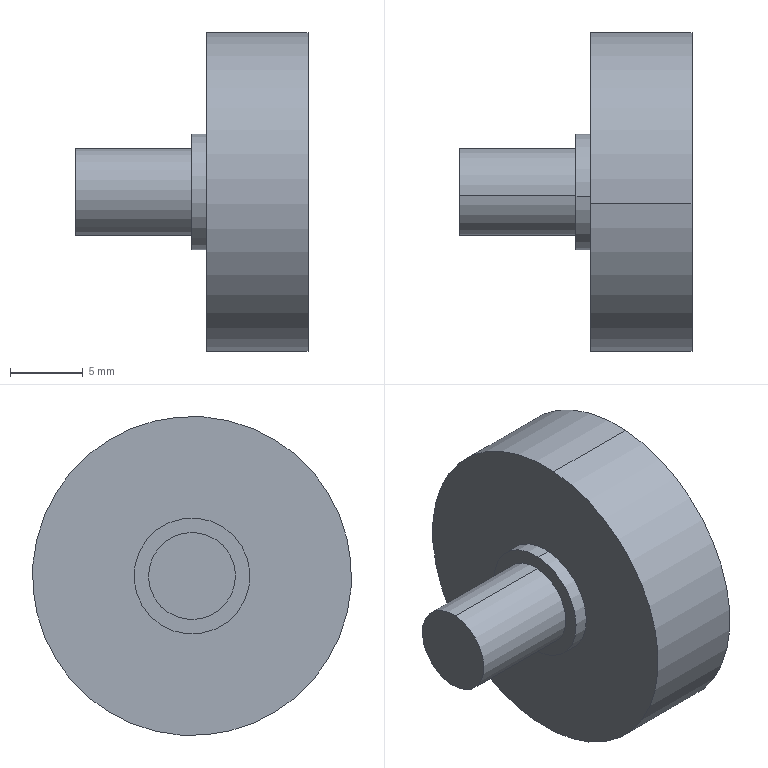Component | SolidWorks | JS60822-7C1L8M6ExternalThreadBearing-1 | 1 solid | 10 faces | box 16 x 22 x 22 mm | volume 2937 mm3 | cylinder 6 | plane 4 | commonest cylinder face diameters 6 x2 8 x2 22 x2
build123d program:
from build123d import *

# Parameters (mm, degrees)
SKETCH1_R           = 11
BOSS_EXTRUDE1_DEPTH = 7
SKETCH2_R           = 4
BOSS_EXTRUDE2_DEPTH = 1
SKETCH3_R           = 3
BOSS_EXTRUDE3_DEPTH = 8


with BuildPart() as part:
    # Sketch1 → Boss-Extrude1 (new body)
    with BuildSketch(Plane(origin=(0, 0, 0), x_dir=(0, 0, -1), z_dir=(1, 0, 0))):
        Circle(SKETCH1_R)
    extrude(amount=BOSS_EXTRUDE1_DEPTH)

    # Sketch2 → Boss-Extrude2 (add)
    with BuildSketch(Plane(origin=(7, 0, 0), x_dir=(0, 0, -1), z_dir=(1, 0, 0))):
        Circle(SKETCH2_R)
    extrude(amount=BOSS_EXTRUDE2_DEPTH)

    # Sketch3 → Boss-Extrude3 (add)
    with BuildSketch(Plane(origin=(8, 0, 0), x_dir=(0, 0, -1), z_dir=(1, 0, 0))):
        Circle(SKETCH3_R)
    extrude(amount=BOSS_EXTRUDE3_DEPTH)


solid = part.part

# Placed as in the assembly
solid = solid.moved(Location((234, 20, 79.212), (-180, 0, 180)))
STEP:
#1=COLOUR_RGB('',0.7922,0.8196,0.9333);
#2=FILL_AREA_STYLE_COLOUR('',#1);
#3=FILL_AREA_STYLE('',(#2));
#4=SURFACE_STYLE_FILL_AREA(#3);
#5=SURFACE_SIDE_STYLE('',(#4));
#6=SURFACE_STYLE_USAGE(.BOTH.,#5);
#7=PRESENTATION_STYLE_ASSIGNMENT((#6));
#8=CARTESIAN_POINT('',(8.583,0.7786,3.236));
#9=VERTEX_POINT('',#8);
#10=CARTESIAN_POINT('',(8.583,0.7962,3.001));
#11=VERTEX_POINT('',#10);
#12=CARTESIAN_POINT('',(8.583,0.7874,3.119));
#13=DIRECTION('',(-1.,-0.,0.));
#14=DIRECTION('',(0.,-0.07456,0.9972));
#15=AXIS2_PLACEMENT_3D('',#12,#13,#14);
#16=CIRCLE('',#15,0.1181);
#17=EDGE_CURVE('',#9,#11,#16,.T.);
#18=ORIENTED_EDGE('',*,*,#17,.F.);
#19=CARTESIAN_POINT('',(8.898,0.7786,3.236));
#20=VERTEX_POINT('',#19);
#21=CARTESIAN_POINT('',(8.583,0.7786,3.236));
#22=DIRECTION('',(1.,0.,0.));
#23=VECTOR('',#22,39.37);
#24=LINE('',#21,#23);
#25=EDGE_CURVE('',#9,#20,#24,.T.);
#26=ORIENTED_EDGE('',*,*,#25,.T.);
#27=CARTESIAN_POINT('',(8.898,0.7962,3.001));
#28=VERTEX_POINT('',#27);
#29=CARTESIAN_POINT('',(8.898,0.7874,3.119));
#30=DIRECTION('',(-1.,-0.,0.));
#31=DIRECTION('',(0.,-0.07456,0.9972));
#32=AXIS2_PLACEMENT_3D('',#29,#30,#31);
#33=CIRCLE('',#32,0.1181);
#34=EDGE_CURVE('',#20,#28,#33,.T.);
#35=ORIENTED_EDGE('',*,*,#34,.T.);
#36=CARTESIAN_POINT('',(8.583,0.7962,3.001));
#37=DIRECTION('',(1.,0.,0.));
#38=VECTOR('',#37,39.37);
#39=LINE('',#36,#38);
#40=EDGE_CURVE('',#11,#28,#39,.T.);
#41=ORIENTED_EDGE('',*,*,#40,.F.);
#42=EDGE_LOOP('',(#18,#26,#35,#41));
#43=FACE_OUTER_BOUND('',#42,.T.);
#44=CARTESIAN_POINT('',(8.583,0.7874,3.119));
#45=DIRECTION('',(1.,0.,0.));
#46=DIRECTION('',(0.,0.07456,-0.9972));
#47=AXIS2_PLACEMENT_3D('',#44,#45,#46);
#48=CYLINDRICAL_SURFACE('',#47,0.1181);
#49=ADVANCED_FACE('',(#43),#48,.T.);
#50=CARTESIAN_POINT('',(8.898,0.7757,3.276));
#51=VERTEX_POINT('',#50);
#52=CARTESIAN_POINT('',(8.898,0.7991,2.962));
#53=VERTEX_POINT('',#52);
#54=CARTESIAN_POINT('',(8.898,0.7874,3.119));
#55=DIRECTION('',(-1.,-0.,0.));
#56=DIRECTION('',(0.,-0.07456,0.9972));
#57=AXIS2_PLACEMENT_3D('',#54,#55,#56);
#58=CIRCLE('',#57,0.1575);
#59=EDGE_CURVE('',#51,#53,#58,.T.);
#60=ORIENTED_EDGE('',*,*,#59,.F.);
#61=CARTESIAN_POINT('',(8.937,0.7757,3.276));
#62=VERTEX_POINT('',#61);
#63=CARTESIAN_POINT('',(8.898,0.7757,3.276));
#64=DIRECTION('',(1.,0.,0.));
#65=VECTOR('',#64,39.37);
#66=LINE('',#63,#65);
#67=EDGE_CURVE('',#51,#62,#66,.T.);
#68=ORIENTED_EDGE('',*,*,#67,.T.);
#69=CARTESIAN_POINT('',(8.937,0.7991,2.962));
#70=VERTEX_POINT('',#69);
#71=CARTESIAN_POINT('',(8.937,0.7874,3.119));
#72=DIRECTION('',(-1.,-0.,0.));
#73=DIRECTION('',(0.,-0.07456,0.9972));
#74=AXIS2_PLACEMENT_3D('',#71,#72,#73);
#75=CIRCLE('',#74,0.1575);
#76=EDGE_CURVE('',#62,#70,#75,.T.);
#77=ORIENTED_EDGE('',*,*,#76,.T.);
#78=CARTESIAN_POINT('',(8.898,0.7991,2.962));
#79=DIRECTION('',(1.,0.,0.));
#80=VECTOR('',#79,39.37);
#81=LINE('',#78,#80);
#82=EDGE_CURVE('',#53,#70,#81,.T.);
#83=ORIENTED_EDGE('',*,*,#82,.F.);
#84=EDGE_LOOP('',(#60,#68,#77,#83));
#85=FACE_OUTER_BOUND('',#84,.T.);
#86=CARTESIAN_POINT('',(8.898,0.7874,3.119));
#87=DIRECTION('',(1.,0.,0.));
#88=DIRECTION('',(0.,0.07456,-0.9972));
#89=AXIS2_PLACEMENT_3D('',#86,#87,#88);
#90=CYLINDRICAL_SURFACE('',#89,0.1575);
#91=ADVANCED_FACE('',(#85),#90,.T.);
#92=CARTESIAN_POINT('',(8.937,0.7551,3.55));
#93=VERTEX_POINT('',#92);
#94=CARTESIAN_POINT('',(8.937,0.8197,2.687));
#95=VERTEX_POINT('',#94);
#96=CARTESIAN_POINT('',(8.937,0.7874,3.119));
#97=DIRECTION('',(-1.,-0.,0.));
#98=DIRECTION('',(0.,-0.07456,0.9972));
#99=AXIS2_PLACEMENT_3D('',#96,#97,#98);
#100=CIRCLE('',#99,0.4331);
#101=EDGE_CURVE('',#93,#95,#100,.T.);
#102=ORIENTED_EDGE('',*,*,#101,.F.);
#103=CARTESIAN_POINT('',(9.213,0.7551,3.55));
#104=VERTEX_POINT('',#103);
#105=CARTESIAN_POINT('',(8.937,0.7551,3.55));
#106=DIRECTION('',(1.,0.,0.));
#107=VECTOR('',#106,39.37);
#108=LINE('',#105,#107);
#109=EDGE_CURVE('',#93,#104,#108,.T.);
#110=ORIENTED_EDGE('',*,*,#109,.T.);
#111=CARTESIAN_POINT('',(9.213,0.8197,2.687));
#112=VERTEX_POINT('',#111);
#113=CARTESIAN_POINT('',(9.213,0.7874,3.119));
#114=DIRECTION('',(-1.,-0.,0.));
#115=DIRECTION('',(0.,-0.07456,0.9972));
#116=AXIS2_PLACEMENT_3D('',#113,#114,#115);
#117=CIRCLE('',#116,0.4331);
#118=EDGE_CURVE('',#104,#112,#117,.T.);
#119=ORIENTED_EDGE('',*,*,#118,.T.);
#120=CARTESIAN_POINT('',(8.937,0.8197,2.687));
#121=DIRECTION('',(1.,0.,0.));
#122=VECTOR('',#121,39.37);
#123=LINE('',#120,#122);
#124=EDGE_CURVE('',#95,#112,#123,.T.);
#125=ORIENTED_EDGE('',*,*,#124,.F.);
#126=EDGE_LOOP('',(#102,#110,#119,#125));
#127=FACE_OUTER_BOUND('',#126,.T.);
#128=CARTESIAN_POINT('',(8.937,0.7874,3.119));
#129=DIRECTION('',(1.,0.,0.));
#130=DIRECTION('',(0.,0.07456,-0.9972));
#131=AXIS2_PLACEMENT_3D('',#128,#129,#130);
#132=CYLINDRICAL_SURFACE('',#131,0.4331);
#133=ADVANCED_FACE('',(#127),#132,.T.);
#134=CARTESIAN_POINT('',(8.898,0.7874,3.119));
#135=DIRECTION('',(-1.,-0.,0.));
#136=DIRECTION('',(0.,-0.07456,0.9972));
#137=AXIS2_PLACEMENT_3D('',#134,#135,#136);
#138=CIRCLE('',#137,0.1575);
#139=EDGE_CURVE('',#53,#51,#138,.T.);
#140=ORIENTED_EDGE('',*,*,#139,.T.);
#141=ORIENTED_EDGE('',*,*,#59,.T.);
#142=EDGE_LOOP('',(#140,#141));
#143=FACE_OUTER_BOUND('',#142,.T.);
#144=CARTESIAN_POINT('',(8.898,0.7874,3.119));
#145=DIRECTION('',(-1.,-0.,0.));
#146=DIRECTION('',(0.,-0.07456,0.9972));
#147=AXIS2_PLACEMENT_3D('',#144,#145,#146);
#148=CIRCLE('',#147,0.1181);
#149=EDGE_CURVE('',#28,#20,#148,.T.);
#150=ORIENTED_EDGE('',*,*,#149,.F.);
#151=ORIENTED_EDGE('',*,*,#34,.F.);
#152=EDGE_LOOP('',(#150,#151));
#153=FACE_BOUND('',#152,.T.);
#154=CARTESIAN_POINT('',(8.898,0.7874,3.119));
#155=DIRECTION('',(-1.,-0.,-0.));
#156=DIRECTION('',(-0.,-0.07456,0.9972));
#157=AXIS2_PLACEMENT_3D('',#154,#155,#156);
#158=PLANE('',#157);
#159=ADVANCED_FACE('',(#143,#153),#158,.T.);
#160=CARTESIAN_POINT('',(8.937,0.7874,3.119));
#161=DIRECTION('',(-1.,-0.,0.));
#162=DIRECTION('',(0.,-0.07456,0.9972));
#163=AXIS2_PLACEMENT_3D('',#160,#161,#162);
#164=CIRCLE('',#163,0.4331);
#165=EDGE_CURVE('',#95,#93,#164,.T.);
#166=ORIENTED_EDGE('',*,*,#165,.T.);
#167=ORIENTED_EDGE('',*,*,#101,.T.);
#168=EDGE_LOOP('',(#166,#167));
#169=FACE_OUTER_BOUND('',#168,.T.);
#170=CARTESIAN_POINT('',(8.937,0.7874,3.119));
#171=DIRECTION('',(-1.,-0.,0.));
#172=DIRECTION('',(0.,-0.07456,0.9972));
#173=AXIS2_PLACEMENT_3D('',#170,#171,#172);
#174=CIRCLE('',#173,0.1575);
#175=EDGE_CURVE('',#70,#62,#174,.T.);
#176=ORIENTED_EDGE('',*,*,#175,.F.);
#177=ORIENTED_EDGE('',*,*,#76,.F.);
#178=EDGE_LOOP('',(#176,#177));
#179=FACE_BOUND('',#178,.T.);
#180=CARTESIAN_POINT('',(8.937,0.7874,3.119));
#181=DIRECTION('',(-1.,-0.,-0.));
#182=DIRECTION('',(-0.,-0.07456,0.9972));
#183=AXIS2_PLACEMENT_3D('',#180,#181,#182);
#184=PLANE('',#183);
#185=ADVANCED_FACE('',(#169,#179),#184,.T.);
#186=ORIENTED_EDGE('',*,*,#109,.F.);
#187=ORIENTED_EDGE('',*,*,#165,.F.);
#188=ORIENTED_EDGE('',*,*,#124,.T.);
#189=CARTESIAN_POINT('',(9.213,0.7874,3.119));
#190=DIRECTION('',(-1.,-0.,0.));
#191=DIRECTION('',(0.,-0.07456,0.9972));
#192=AXIS2_PLACEMENT_3D('',#189,#190,#191);
#193=CIRCLE('',#192,0.4331);
#194=EDGE_CURVE('',#112,#104,#193,.T.);
#195=ORIENTED_EDGE('',*,*,#194,.T.);
#196=EDGE_LOOP('',(#186,#187,#188,#195));
#197=FACE_OUTER_BOUND('',#196,.T.);
#198=CARTESIAN_POINT('',(8.937,0.7874,3.119));
#199=DIRECTION('',(1.,0.,0.));
#200=DIRECTION('',(0.,0.07456,-0.9972));
#201=AXIS2_PLACEMENT_3D('',#198,#199,#200);
#202=CYLINDRICAL_SURFACE('',#201,0.4331);
#203=ADVANCED_FACE('',(#197),#202,.T.);
#204=ORIENTED_EDGE('',*,*,#194,.F.);
#205=ORIENTED_EDGE('',*,*,#118,.F.);
#206=EDGE_LOOP('',(#204,#205));
#207=FACE_OUTER_BOUND('',#206,.T.);
#208=CARTESIAN_POINT('',(9.213,0.7874,3.119));
#209=DIRECTION('',(-1.,-0.,-0.));
#210=DIRECTION('',(-0.,-0.07456,0.9972));
#211=AXIS2_PLACEMENT_3D('',#208,#209,#210);
#212=PLANE('',#211);
#213=ADVANCED_FACE('',(#207),#212,.F.);
#214=ORIENTED_EDGE('',*,*,#67,.F.);
#215=ORIENTED_EDGE('',*,*,#139,.F.);
#216=ORIENTED_EDGE('',*,*,#82,.T.);
#217=ORIENTED_EDGE('',*,*,#175,.T.);
#218=EDGE_LOOP('',(#214,#215,#216,#217));
#219=FACE_OUTER_BOUND('',#218,.T.);
#220=CARTESIAN_POINT('',(8.898,0.7874,3.119));
#221=DIRECTION('',(1.,0.,0.));
#222=DIRECTION('',(0.,0.07456,-0.9972));
#223=AXIS2_PLACEMENT_3D('',#220,#221,#222);
#224=CYLINDRICAL_SURFACE('',#223,0.1575);
#225=ADVANCED_FACE('',(#219),#224,.T.);
#226=ORIENTED_EDGE('',*,*,#25,.F.);
#227=CARTESIAN_POINT('',(8.583,0.7874,3.119));
#228=DIRECTION('',(-1.,-0.,0.));
#229=DIRECTION('',(0.,-0.07456,0.9972));
#230=AXIS2_PLACEMENT_3D('',#227,#228,#229);
#231=CIRCLE('',#230,0.1181);
#232=EDGE_CURVE('',#11,#9,#231,.T.);
#233=ORIENTED_EDGE('',*,*,#232,.F.);
#234=ORIENTED_EDGE('',*,*,#40,.T.);
#235=ORIENTED_EDGE('',*,*,#149,.T.);
#236=EDGE_LOOP('',(#226,#233,#234,#235));
#237=FACE_OUTER_BOUND('',#236,.T.);
#238=CARTESIAN_POINT('',(8.583,0.7874,3.119));
#239=DIRECTION('',(1.,0.,0.));
#240=DIRECTION('',(0.,0.07456,-0.9972));
#241=AXIS2_PLACEMENT_3D('',#238,#239,#240);
#242=CYLINDRICAL_SURFACE('',#241,0.1181);
#243=ADVANCED_FACE('',(#237),#242,.T.);
#244=ORIENTED_EDGE('',*,*,#232,.T.);
#245=ORIENTED_EDGE('',*,*,#17,.T.);
#246=EDGE_LOOP('',(#244,#245));
#247=FACE_OUTER_BOUND('',#246,.T.);
#248=CARTESIAN_POINT('',(8.583,0.7874,3.119));
#249=DIRECTION('',(-1.,-0.,-0.));
#250=DIRECTION('',(-0.,-0.07456,0.9972));
#251=AXIS2_PLACEMENT_3D('',#248,#249,#250);
#252=PLANE('',#251);
#253=ADVANCED_FACE('',(#247),#252,.T.);
#254=CLOSED_SHELL('',(#49,#91,#133,#159,#185,#203,#213,#225,#243,#253));
#255=MANIFOLD_SOLID_BREP('',#254);
#256=STYLED_ITEM('',(#7),#255);
#257=PRESENTATION_LAYER_ASSIGNMENT('','',(#256));
#258=(LENGTH_UNIT()NAMED_UNIT(*)SI_UNIT($,.METRE.));
#259=LENGTH_MEASURE_WITH_UNIT(LENGTH_MEASURE(0.0254),#258);
#260=DIMENSIONAL_EXPONENTS(1.,0.,0.,0.,0.,0.,0.);
#261=(CONVERSION_BASED_UNIT('',#259)LENGTH_UNIT()NAMED_UNIT(#260));
#262=UNCERTAINTY_MEASURE_WITH_UNIT(LENGTH_MEASURE(0.00001),#261,'','');
#263=(NAMED_UNIT(*)PLANE_ANGLE_UNIT()SI_UNIT($,.RADIAN.));
#264=(NAMED_UNIT(*)SI_UNIT($,.STERADIAN.)SOLID_ANGLE_UNIT());
#265=(GEOMETRIC_REPRESENTATION_CONTEXT(3)GLOBAL_UNCERTAINTY_ASSIGNED_CONTEXT((#262))GLOBAL_UNIT_ASSIGNED_CONTEXT((#261,#263,#264))REPRESENTATION_CONTEXT('',''));
#266=MECHANICAL_DESIGN_GEOMETRIC_PRESENTATION_REPRESENTATION('',(#256),#265);
#267=CARTESIAN_POINT('',(0.,0.,0.));
#268=DIRECTION('',(0.,0.,1.));
#269=DIRECTION('',(1.,0.,0.));
#270=AXIS2_PLACEMENT_3D('',#267,#268,#269);
#271=(LENGTH_UNIT()NAMED_UNIT(*)SI_UNIT($,.METRE.));
#272=LENGTH_MEASURE_WITH_UNIT(LENGTH_MEASURE(0.0254),#271);
#273=DIMENSIONAL_EXPONENTS(1.,0.,0.,0.,0.,0.,0.);
#274=(CONVERSION_BASED_UNIT('',#272)LENGTH_UNIT()NAMED_UNIT(#273));
#275=UNCERTAINTY_MEASURE_WITH_UNIT(LENGTH_MEASURE(0.00001),#274,'','');
#276=(NAMED_UNIT(*)PLANE_ANGLE_UNIT()SI_UNIT($,.RADIAN.));
#277=(NAMED_UNIT(*)SI_UNIT($,.STERADIAN.)SOLID_ANGLE_UNIT());
#278=(GEOMETRIC_REPRESENTATION_CONTEXT(3)GLOBAL_UNCERTAINTY_ASSIGNED_CONTEXT((#275))GLOBAL_UNIT_ASSIGNED_CONTEXT((#274,#276,#277))REPRESENTATION_CONTEXT('',''));
#279=ADVANCED_BREP_SHAPE_REPRESENTATION('',(#255,#270),#278);